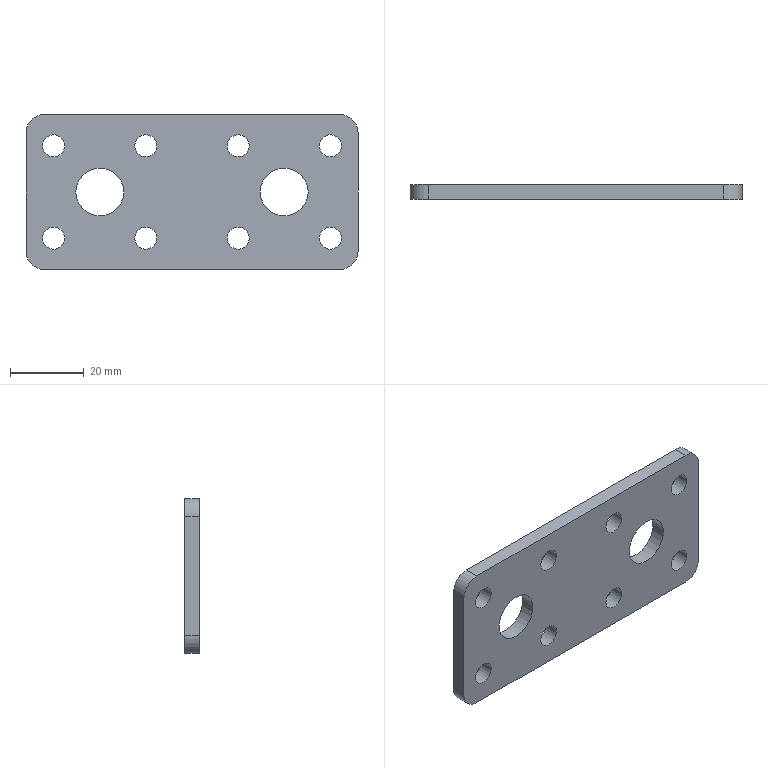Component | SolidWorks | ConnectingPlate(No.9)-3 | 1 solid | 30 faces | box 90 x 4 x 42 mm | volume 13068 mm3 | cylinder 24 | plane 6 | commonest cylinder face diameters 6 x16 13 x4 10 x4 | material Plain Carbon Steel
STEP:
#1=CARTESIAN_POINT('',(12.185,-14.764,-0.4921));
#2=VERTEX_POINT('',#1);
#3=CARTESIAN_POINT('',(12.421,-14.764,-0.4921));
#4=VERTEX_POINT('',#3);
#5=CARTESIAN_POINT('',(12.303,-14.764,-0.4921));
#6=DIRECTION('',(-0.,1.,0.));
#7=DIRECTION('',(-1.,0.,0.));
#8=AXIS2_PLACEMENT_3D('',#5,#6,#7);
#9=CIRCLE('',#8,0.1181);
#10=EDGE_CURVE('',#2,#4,#9,.T.);
#11=ORIENTED_EDGE('',*,*,#10,.F.);
#12=CARTESIAN_POINT('',(12.185,-14.606,-0.4921));
#13=VERTEX_POINT('',#12);
#14=CARTESIAN_POINT('',(12.185,-14.764,-0.4921));
#15=DIRECTION('',(-0.,1.,0.));
#16=VECTOR('',#15,39.37);
#17=LINE('',#14,#16);
#18=EDGE_CURVE('',#2,#13,#17,.T.);
#19=ORIENTED_EDGE('',*,*,#18,.T.);
#20=CARTESIAN_POINT('',(12.421,-14.606,-0.4921));
#21=VERTEX_POINT('',#20);
#22=CARTESIAN_POINT('',(12.303,-14.606,-0.4921));
#23=DIRECTION('',(-0.,1.,0.));
#24=DIRECTION('',(-1.,0.,0.));
#25=AXIS2_PLACEMENT_3D('',#22,#23,#24);
#26=CIRCLE('',#25,0.1181);
#27=EDGE_CURVE('',#13,#21,#26,.T.);
#28=ORIENTED_EDGE('',*,*,#27,.T.);
#29=CARTESIAN_POINT('',(12.421,-14.764,-0.4921));
#30=DIRECTION('',(-0.,1.,0.));
#31=VECTOR('',#30,39.37);
#32=LINE('',#29,#31);
#33=EDGE_CURVE('',#4,#21,#32,.T.);
#34=ORIENTED_EDGE('',*,*,#33,.F.);
#35=EDGE_LOOP('',(#11,#19,#28,#34));
#36=FACE_OUTER_BOUND('',#35,.T.);
#37=CARTESIAN_POINT('',(12.303,-14.764,-0.4921));
#38=DIRECTION('',(-0.,1.,0.));
#39=DIRECTION('',(1.,0.,-0.));
#40=AXIS2_PLACEMENT_3D('',#37,#38,#39);
#41=CYLINDRICAL_SURFACE('',#40,0.1181);
#42=ADVANCED_FACE('',(#36),#41,.F.);
#43=CARTESIAN_POINT('',(13.169,-14.764,-0.4921));
#44=VERTEX_POINT('',#43);
#45=CARTESIAN_POINT('',(13.406,-14.764,-0.4921));
#46=VERTEX_POINT('',#45);
#47=CARTESIAN_POINT('',(13.287,-14.764,-0.4921));
#48=DIRECTION('',(-0.,1.,0.));
#49=DIRECTION('',(-1.,0.,0.));
#50=AXIS2_PLACEMENT_3D('',#47,#48,#49);
#51=CIRCLE('',#50,0.1181);
#52=EDGE_CURVE('',#44,#46,#51,.T.);
#53=ORIENTED_EDGE('',*,*,#52,.F.);
#54=CARTESIAN_POINT('',(13.169,-14.606,-0.4921));
#55=VERTEX_POINT('',#54);
#56=CARTESIAN_POINT('',(13.169,-14.764,-0.4921));
#57=DIRECTION('',(-0.,1.,0.));
#58=VECTOR('',#57,39.37);
#59=LINE('',#56,#58);
#60=EDGE_CURVE('',#44,#55,#59,.T.);
#61=ORIENTED_EDGE('',*,*,#60,.T.);
#62=CARTESIAN_POINT('',(13.406,-14.606,-0.4921));
#63=VERTEX_POINT('',#62);
#64=CARTESIAN_POINT('',(13.287,-14.606,-0.4921));
#65=DIRECTION('',(-0.,1.,0.));
#66=DIRECTION('',(-1.,0.,0.));
#67=AXIS2_PLACEMENT_3D('',#64,#65,#66);
#68=CIRCLE('',#67,0.1181);
#69=EDGE_CURVE('',#55,#63,#68,.T.);
#70=ORIENTED_EDGE('',*,*,#69,.T.);
#71=CARTESIAN_POINT('',(13.406,-14.764,-0.4921));
#72=DIRECTION('',(-0.,1.,0.));
#73=VECTOR('',#72,39.37);
#74=LINE('',#71,#73);
#75=EDGE_CURVE('',#46,#63,#74,.T.);
#76=ORIENTED_EDGE('',*,*,#75,.F.);
#77=EDGE_LOOP('',(#53,#61,#70,#76));
#78=FACE_OUTER_BOUND('',#77,.T.);
#79=CARTESIAN_POINT('',(13.287,-14.764,-0.4921));
#80=DIRECTION('',(-0.,1.,0.));
#81=DIRECTION('',(1.,0.,-0.));
#82=AXIS2_PLACEMENT_3D('',#79,#80,#81);
#83=CYLINDRICAL_SURFACE('',#82,0.1181);
#84=ADVANCED_FACE('',(#78),#83,.F.);
#85=CARTESIAN_POINT('',(14.154,-14.764,-0.4921));
#86=VERTEX_POINT('',#85);
#87=CARTESIAN_POINT('',(14.39,-14.764,-0.4921));
#88=VERTEX_POINT('',#87);
#89=CARTESIAN_POINT('',(14.272,-14.764,-0.4921));
#90=DIRECTION('',(-0.,1.,0.));
#91=DIRECTION('',(-1.,0.,0.));
#92=AXIS2_PLACEMENT_3D('',#89,#90,#91);
#93=CIRCLE('',#92,0.1181);
#94=EDGE_CURVE('',#86,#88,#93,.T.);
#95=ORIENTED_EDGE('',*,*,#94,.F.);
#96=CARTESIAN_POINT('',(14.154,-14.606,-0.4921));
#97=VERTEX_POINT('',#96);
#98=CARTESIAN_POINT('',(14.154,-14.764,-0.4921));
#99=DIRECTION('',(-0.,1.,0.));
#100=VECTOR('',#99,39.37);
#101=LINE('',#98,#100);
#102=EDGE_CURVE('',#86,#97,#101,.T.);
#103=ORIENTED_EDGE('',*,*,#102,.T.);
#104=CARTESIAN_POINT('',(14.39,-14.606,-0.4921));
#105=VERTEX_POINT('',#104);
#106=CARTESIAN_POINT('',(14.272,-14.606,-0.4921));
#107=DIRECTION('',(-0.,1.,0.));
#108=DIRECTION('',(-1.,0.,0.));
#109=AXIS2_PLACEMENT_3D('',#106,#107,#108);
#110=CIRCLE('',#109,0.1181);
#111=EDGE_CURVE('',#97,#105,#110,.T.);
#112=ORIENTED_EDGE('',*,*,#111,.T.);
#113=CARTESIAN_POINT('',(14.39,-14.764,-0.4921));
#114=DIRECTION('',(-0.,1.,0.));
#115=VECTOR('',#114,39.37);
#116=LINE('',#113,#115);
#117=EDGE_CURVE('',#88,#105,#116,.T.);
#118=ORIENTED_EDGE('',*,*,#117,.F.);
#119=EDGE_LOOP('',(#95,#103,#112,#118));
#120=FACE_OUTER_BOUND('',#119,.T.);
#121=CARTESIAN_POINT('',(14.272,-14.764,-0.4921));
#122=DIRECTION('',(-0.,1.,0.));
#123=DIRECTION('',(1.,0.,-0.));
#124=AXIS2_PLACEMENT_3D('',#121,#122,#123);
#125=CYLINDRICAL_SURFACE('',#124,0.1181);
#126=ADVANCED_FACE('',(#120),#125,.F.);
#127=CARTESIAN_POINT('',(15.138,-14.764,-0.4921));
#128=VERTEX_POINT('',#127);
#129=CARTESIAN_POINT('',(15.374,-14.764,-0.4921));
#130=VERTEX_POINT('',#129);
#131=CARTESIAN_POINT('',(15.256,-14.764,-0.4921));
#132=DIRECTION('',(-0.,1.,0.));
#133=DIRECTION('',(-1.,0.,0.));
#134=AXIS2_PLACEMENT_3D('',#131,#132,#133);
#135=CIRCLE('',#134,0.1181);
#136=EDGE_CURVE('',#128,#130,#135,.T.);
#137=ORIENTED_EDGE('',*,*,#136,.F.);
#138=CARTESIAN_POINT('',(15.138,-14.606,-0.4921));
#139=VERTEX_POINT('',#138);
#140=CARTESIAN_POINT('',(15.138,-14.764,-0.4921));
#141=DIRECTION('',(-0.,1.,0.));
#142=VECTOR('',#141,39.37);
#143=LINE('',#140,#142);
#144=EDGE_CURVE('',#128,#139,#143,.T.);
#145=ORIENTED_EDGE('',*,*,#144,.T.);
#146=CARTESIAN_POINT('',(15.374,-14.606,-0.4921));
#147=VERTEX_POINT('',#146);
#148=CARTESIAN_POINT('',(15.256,-14.606,-0.4921));
#149=DIRECTION('',(-0.,1.,0.));
#150=DIRECTION('',(-1.,0.,0.));
#151=AXIS2_PLACEMENT_3D('',#148,#149,#150);
#152=CIRCLE('',#151,0.1181);
#153=EDGE_CURVE('',#139,#147,#152,.T.);
#154=ORIENTED_EDGE('',*,*,#153,.T.);
#155=CARTESIAN_POINT('',(15.374,-14.764,-0.4921));
#156=DIRECTION('',(-0.,1.,0.));
#157=VECTOR('',#156,39.37);
#158=LINE('',#155,#157);
#159=EDGE_CURVE('',#130,#147,#158,.T.);
#160=ORIENTED_EDGE('',*,*,#159,.F.);
#161=EDGE_LOOP('',(#137,#145,#154,#160));
#162=FACE_OUTER_BOUND('',#161,.T.);
#163=CARTESIAN_POINT('',(15.256,-14.764,-0.4921));
#164=DIRECTION('',(-0.,1.,0.));
#165=DIRECTION('',(1.,0.,-0.));
#166=AXIS2_PLACEMENT_3D('',#163,#164,#165);
#167=CYLINDRICAL_SURFACE('',#166,0.1181);
#168=ADVANCED_FACE('',(#162),#167,.F.);
#169=CARTESIAN_POINT('',(15.138,-14.764,-1.476));
#170=VERTEX_POINT('',#169);
#171=CARTESIAN_POINT('',(15.374,-14.764,-1.476));
#172=VERTEX_POINT('',#171);
#173=CARTESIAN_POINT('',(15.256,-14.764,-1.476));
#174=DIRECTION('',(-0.,1.,0.));
#175=DIRECTION('',(1.,0.,0.));
#176=AXIS2_PLACEMENT_3D('',#173,#174,#175);
#177=CIRCLE('',#176,0.1181);
#178=EDGE_CURVE('',#170,#172,#177,.T.);
#179=ORIENTED_EDGE('',*,*,#178,.F.);
#180=CARTESIAN_POINT('',(15.138,-14.606,-1.476));
#181=VERTEX_POINT('',#180);
#182=CARTESIAN_POINT('',(15.138,-14.764,-1.476));
#183=DIRECTION('',(-0.,1.,0.));
#184=VECTOR('',#183,39.37);
#185=LINE('',#182,#184);
#186=EDGE_CURVE('',#170,#181,#185,.T.);
#187=ORIENTED_EDGE('',*,*,#186,.T.);
#188=CARTESIAN_POINT('',(15.374,-14.606,-1.476));
#189=VERTEX_POINT('',#188);
#190=CARTESIAN_POINT('',(15.256,-14.606,-1.476));
#191=DIRECTION('',(-0.,1.,0.));
#192=DIRECTION('',(1.,0.,0.));
#193=AXIS2_PLACEMENT_3D('',#190,#191,#192);
#194=CIRCLE('',#193,0.1181);
#195=EDGE_CURVE('',#181,#189,#194,.T.);
#196=ORIENTED_EDGE('',*,*,#195,.T.);
#197=CARTESIAN_POINT('',(15.374,-14.764,-1.476));
#198=DIRECTION('',(-0.,1.,0.));
#199=VECTOR('',#198,39.37);
#200=LINE('',#197,#199);
#201=EDGE_CURVE('',#172,#189,#200,.T.);
#202=ORIENTED_EDGE('',*,*,#201,.F.);
#203=EDGE_LOOP('',(#179,#187,#196,#202));
#204=FACE_OUTER_BOUND('',#203,.T.);
#205=CARTESIAN_POINT('',(15.256,-14.764,-1.476));
#206=DIRECTION('',(-0.,1.,0.));
#207=DIRECTION('',(1.,0.,0.));
#208=AXIS2_PLACEMENT_3D('',#205,#206,#207);
#209=CYLINDRICAL_SURFACE('',#208,0.1181);
#210=ADVANCED_FACE('',(#204),#209,.F.);
#211=CARTESIAN_POINT('',(14.154,-14.764,-1.476));
#212=VERTEX_POINT('',#211);
#213=CARTESIAN_POINT('',(14.39,-14.764,-1.476));
#214=VERTEX_POINT('',#213);
#215=CARTESIAN_POINT('',(14.272,-14.764,-1.476));
#216=DIRECTION('',(-0.,1.,0.));
#217=DIRECTION('',(1.,0.,0.));
#218=AXIS2_PLACEMENT_3D('',#215,#216,#217);
#219=CIRCLE('',#218,0.1181);
#220=EDGE_CURVE('',#212,#214,#219,.T.);
#221=ORIENTED_EDGE('',*,*,#220,.F.);
#222=CARTESIAN_POINT('',(14.154,-14.606,-1.476));
#223=VERTEX_POINT('',#222);
#224=CARTESIAN_POINT('',(14.154,-14.764,-1.476));
#225=DIRECTION('',(-0.,1.,0.));
#226=VECTOR('',#225,39.37);
#227=LINE('',#224,#226);
#228=EDGE_CURVE('',#212,#223,#227,.T.);
#229=ORIENTED_EDGE('',*,*,#228,.T.);
#230=CARTESIAN_POINT('',(14.39,-14.606,-1.476));
#231=VERTEX_POINT('',#230);
#232=CARTESIAN_POINT('',(14.272,-14.606,-1.476));
#233=DIRECTION('',(-0.,1.,0.));
#234=DIRECTION('',(1.,0.,0.));
#235=AXIS2_PLACEMENT_3D('',#232,#233,#234);
#236=CIRCLE('',#235,0.1181);
#237=EDGE_CURVE('',#223,#231,#236,.T.);
#238=ORIENTED_EDGE('',*,*,#237,.T.);
#239=CARTESIAN_POINT('',(14.39,-14.764,-1.476));
#240=DIRECTION('',(-0.,1.,0.));
#241=VECTOR('',#240,39.37);
#242=LINE('',#239,#241);
#243=EDGE_CURVE('',#214,#231,#242,.T.);
#244=ORIENTED_EDGE('',*,*,#243,.F.);
#245=EDGE_LOOP('',(#221,#229,#238,#244));
#246=FACE_OUTER_BOUND('',#245,.T.);
#247=CARTESIAN_POINT('',(14.272,-14.764,-1.476));
#248=DIRECTION('',(-0.,1.,0.));
#249=DIRECTION('',(1.,0.,0.));
#250=AXIS2_PLACEMENT_3D('',#247,#248,#249);
#251=CYLINDRICAL_SURFACE('',#250,0.1181);
#252=ADVANCED_FACE('',(#246),#251,.F.);
#253=CARTESIAN_POINT('',(13.169,-14.764,-1.476));
#254=VERTEX_POINT('',#253);
#255=CARTESIAN_POINT('',(13.406,-14.764,-1.476));
#256=VERTEX_POINT('',#255);
#257=CARTESIAN_POINT('',(13.287,-14.764,-1.476));
#258=DIRECTION('',(-0.,1.,0.));
#259=DIRECTION('',(1.,0.,0.));
#260=AXIS2_PLACEMENT_3D('',#257,#258,#259);
#261=CIRCLE('',#260,0.1181);
#262=EDGE_CURVE('',#254,#256,#261,.T.);
#263=ORIENTED_EDGE('',*,*,#262,.F.);
#264=CARTESIAN_POINT('',(13.169,-14.606,-1.476));
#265=VERTEX_POINT('',#264);
#266=CARTESIAN_POINT('',(13.169,-14.764,-1.476));
#267=DIRECTION('',(-0.,1.,0.));
#268=VECTOR('',#267,39.37);
#269=LINE('',#266,#268);
#270=EDGE_CURVE('',#254,#265,#269,.T.);
#271=ORIENTED_EDGE('',*,*,#270,.T.);
#272=CARTESIAN_POINT('',(13.406,-14.606,-1.476));
#273=VERTEX_POINT('',#272);
#274=CARTESIAN_POINT('',(13.287,-14.606,-1.476));
#275=DIRECTION('',(-0.,1.,0.));
#276=DIRECTION('',(1.,0.,0.));
#277=AXIS2_PLACEMENT_3D('',#274,#275,#276);
#278=CIRCLE('',#277,0.1181);
#279=EDGE_CURVE('',#265,#273,#278,.T.);
#280=ORIENTED_EDGE('',*,*,#279,.T.);
#281=CARTESIAN_POINT('',(13.406,-14.764,-1.476));
#282=DIRECTION('',(-0.,1.,0.));
#283=VECTOR('',#282,39.37);
#284=LINE('',#281,#283);
#285=EDGE_CURVE('',#256,#273,#284,.T.);
#286=ORIENTED_EDGE('',*,*,#285,.F.);
#287=EDGE_LOOP('',(#263,#271,#280,#286));
#288=FACE_OUTER_BOUND('',#287,.T.);
#289=CARTESIAN_POINT('',(13.287,-14.764,-1.476));
#290=DIRECTION('',(-0.,1.,0.));
#291=DIRECTION('',(1.,0.,0.));
#292=AXIS2_PLACEMENT_3D('',#289,#290,#291);
#293=CYLINDRICAL_SURFACE('',#292,0.1181);
#294=ADVANCED_FACE('',(#288),#293,.F.);
#295=CARTESIAN_POINT('',(12.185,-14.764,-1.476));
#296=VERTEX_POINT('',#295);
#297=CARTESIAN_POINT('',(12.421,-14.764,-1.476));
#298=VERTEX_POINT('',#297);
#299=CARTESIAN_POINT('',(12.303,-14.764,-1.476));
#300=DIRECTION('',(-0.,1.,0.));
#301=DIRECTION('',(1.,0.,0.));
#302=AXIS2_PLACEMENT_3D('',#299,#300,#301);
#303=CIRCLE('',#302,0.1181);
#304=EDGE_CURVE('',#296,#298,#303,.T.);
#305=ORIENTED_EDGE('',*,*,#304,.F.);
#306=CARTESIAN_POINT('',(12.185,-14.606,-1.476));
#307=VERTEX_POINT('',#306);
#308=CARTESIAN_POINT('',(12.185,-14.764,-1.476));
#309=DIRECTION('',(-0.,1.,0.));
#310=VECTOR('',#309,39.37);
#311=LINE('',#308,#310);
#312=EDGE_CURVE('',#296,#307,#311,.T.);
#313=ORIENTED_EDGE('',*,*,#312,.T.);
#314=CARTESIAN_POINT('',(12.421,-14.606,-1.476));
#315=VERTEX_POINT('',#314);
#316=CARTESIAN_POINT('',(12.303,-14.606,-1.476));
#317=DIRECTION('',(-0.,1.,0.));
#318=DIRECTION('',(1.,0.,0.));
#319=AXIS2_PLACEMENT_3D('',#316,#317,#318);
#320=CIRCLE('',#319,0.1181);
#321=EDGE_CURVE('',#307,#315,#320,.T.);
#322=ORIENTED_EDGE('',*,*,#321,.T.);
#323=CARTESIAN_POINT('',(12.421,-14.764,-1.476));
#324=DIRECTION('',(-0.,1.,0.));
#325=VECTOR('',#324,39.37);
#326=LINE('',#323,#325);
#327=EDGE_CURVE('',#298,#315,#326,.T.);
#328=ORIENTED_EDGE('',*,*,#327,.F.);
#329=EDGE_LOOP('',(#305,#313,#322,#328));
#330=FACE_OUTER_BOUND('',#329,.T.);
#331=CARTESIAN_POINT('',(12.303,-14.764,-1.476));
#332=DIRECTION('',(-0.,1.,0.));
#333=DIRECTION('',(1.,0.,0.));
#334=AXIS2_PLACEMENT_3D('',#331,#332,#333);
#335=CYLINDRICAL_SURFACE('',#334,0.1181);
#336=ADVANCED_FACE('',(#330),#335,.F.);
#337=CARTESIAN_POINT('',(14.508,-14.764,-0.9843));
#338=VERTEX_POINT('',#337);
#339=CARTESIAN_POINT('',(15.02,-14.764,-0.9843));
#340=VERTEX_POINT('',#339);
#341=CARTESIAN_POINT('',(14.764,-14.764,-0.9843));
#342=DIRECTION('',(-0.,1.,0.));
#343=DIRECTION('',(-1.,0.,0.));
#344=AXIS2_PLACEMENT_3D('',#341,#342,#343);
#345=CIRCLE('',#344,0.2559);
#346=EDGE_CURVE('',#338,#340,#345,.T.);
#347=ORIENTED_EDGE('',*,*,#346,.F.);
#348=CARTESIAN_POINT('',(14.508,-14.606,-0.9843));
#349=VERTEX_POINT('',#348);
#350=CARTESIAN_POINT('',(14.508,-14.764,-0.9843));
#351=DIRECTION('',(-0.,1.,0.));
#352=VECTOR('',#351,39.37);
#353=LINE('',#350,#352);
#354=EDGE_CURVE('',#338,#349,#353,.T.);
#355=ORIENTED_EDGE('',*,*,#354,.T.);
#356=CARTESIAN_POINT('',(15.02,-14.606,-0.9843));
#357=VERTEX_POINT('',#356);
#358=CARTESIAN_POINT('',(14.764,-14.606,-0.9843));
#359=DIRECTION('',(-0.,1.,0.));
#360=DIRECTION('',(-1.,0.,0.));
#361=AXIS2_PLACEMENT_3D('',#358,#359,#360);
#362=CIRCLE('',#361,0.2559);
#363=EDGE_CURVE('',#349,#357,#362,.T.);
#364=ORIENTED_EDGE('',*,*,#363,.T.);
#365=CARTESIAN_POINT('',(15.02,-14.764,-0.9843));
#366=DIRECTION('',(-0.,1.,0.));
#367=VECTOR('',#366,39.37);
#368=LINE('',#365,#367);
#369=EDGE_CURVE('',#340,#357,#368,.T.);
#370=ORIENTED_EDGE('',*,*,#369,.F.);
#371=EDGE_LOOP('',(#347,#355,#364,#370));
#372=FACE_OUTER_BOUND('',#371,.T.);
#373=CARTESIAN_POINT('',(14.764,-14.764,-0.9843));
#374=DIRECTION('',(-0.,1.,0.));
#375=DIRECTION('',(1.,0.,-0.));
#376=AXIS2_PLACEMENT_3D('',#373,#374,#375);
#377=CYLINDRICAL_SURFACE('',#376,0.2559);
#378=ADVANCED_FACE('',(#372),#377,.F.);
#379=CARTESIAN_POINT('',(12.539,-14.764,-0.9843));
#380=VERTEX_POINT('',#379);
#381=CARTESIAN_POINT('',(13.051,-14.764,-0.9843));
#382=VERTEX_POINT('',#381);
#383=CARTESIAN_POINT('',(12.795,-14.764,-0.9843));
#384=DIRECTION('',(-0.,1.,0.));
#385=DIRECTION('',(1.,0.,-0.));
#386=AXIS2_PLACEMENT_3D('',#383,#384,#385);
#387=CIRCLE('',#386,0.2559);
#388=EDGE_CURVE('',#380,#382,#387,.T.);
#389=ORIENTED_EDGE('',*,*,#388,.F.);
#390=CARTESIAN_POINT('',(12.539,-14.606,-0.9843));
#391=VERTEX_POINT('',#390);
#392=CARTESIAN_POINT('',(12.539,-14.764,-0.9843));
#393=DIRECTION('',(-0.,1.,0.));
#394=VECTOR('',#393,39.37);
#395=LINE('',#392,#394);
#396=EDGE_CURVE('',#380,#391,#395,.T.);
#397=ORIENTED_EDGE('',*,*,#396,.T.);
#398=CARTESIAN_POINT('',(13.051,-14.606,-0.9843));
#399=VERTEX_POINT('',#398);
#400=CARTESIAN_POINT('',(12.795,-14.606,-0.9843));
#401=DIRECTION('',(-0.,1.,0.));
#402=DIRECTION('',(1.,0.,-0.));
#403=AXIS2_PLACEMENT_3D('',#400,#401,#402);
#404=CIRCLE('',#403,0.2559);
#405=EDGE_CURVE('',#391,#399,#404,.T.);
#406=ORIENTED_EDGE('',*,*,#405,.T.);
#407=CARTESIAN_POINT('',(13.051,-14.764,-0.9843));
#408=DIRECTION('',(-0.,1.,0.));
#409=VECTOR('',#408,39.37);
#410=LINE('',#407,#409);
#411=EDGE_CURVE('',#382,#399,#410,.T.);
#412=ORIENTED_EDGE('',*,*,#411,.F.);
#413=EDGE_LOOP('',(#389,#397,#406,#412));
#414=FACE_OUTER_BOUND('',#413,.T.);
#415=CARTESIAN_POINT('',(12.795,-14.764,-0.9843));
#416=DIRECTION('',(-0.,1.,0.));
#417=DIRECTION('',(1.,0.,-0.));
#418=AXIS2_PLACEMENT_3D('',#415,#416,#417);
#419=CYLINDRICAL_SURFACE('',#418,0.2559);
#420=ADVANCED_FACE('',(#414),#419,.F.);
#421=CARTESIAN_POINT('',(15.551,-14.606,-0.3543));
#422=VERTEX_POINT('',#421);
#423=CARTESIAN_POINT('',(15.551,-14.606,-1.614));
#424=VERTEX_POINT('',#423);
#425=CARTESIAN_POINT('',(15.551,-14.606,-0.1575));
#426=DIRECTION('',(-0.,0.,-1.));
#427=VECTOR('',#426,39.37);
#428=LINE('',#425,#427);
#429=EDGE_CURVE('',#422,#424,#428,.T.);
#430=ORIENTED_EDGE('',*,*,#429,.F.);
#431=CARTESIAN_POINT('',(15.551,-14.764,-0.3543));
#432=VERTEX_POINT('',#431);
#433=CARTESIAN_POINT('',(15.551,-14.764,-0.3543));
#434=DIRECTION('',(0.,-1.,-0.));
#435=VECTOR('',#434,39.37);
#436=LINE('',#433,#435);
#437=EDGE_CURVE('',#422,#432,#436,.T.);
#438=ORIENTED_EDGE('',*,*,#437,.T.);
#439=CARTESIAN_POINT('',(15.551,-14.764,-1.614));
#440=VERTEX_POINT('',#439);
#441=CARTESIAN_POINT('',(15.551,-14.764,-0.1575));
#442=DIRECTION('',(-0.,0.,-1.));
#443=VECTOR('',#442,39.37);
#444=LINE('',#441,#443);
#445=EDGE_CURVE('',#432,#440,#444,.T.);
#446=ORIENTED_EDGE('',*,*,#445,.T.);
#447=CARTESIAN_POINT('',(15.551,-14.764,-1.614));
#448=DIRECTION('',(-0.,1.,0.));
#449=VECTOR('',#448,39.37);
#450=LINE('',#447,#449);
#451=EDGE_CURVE('',#440,#424,#450,.T.);
#452=ORIENTED_EDGE('',*,*,#451,.T.);
#453=EDGE_LOOP('',(#430,#438,#446,#452));
#454=FACE_OUTER_BOUND('',#453,.T.);
#455=CARTESIAN_POINT('',(15.551,-14.764,-0.1575));
#456=DIRECTION('',(1.,0.,-0.));
#457=DIRECTION('',(0.,-1.,-0.));
#458=AXIS2_PLACEMENT_3D('',#455,#456,#457);
#459=PLANE('',#458);
#460=ADVANCED_FACE('',(#454),#459,.T.);
#461=CARTESIAN_POINT('',(12.205,-14.606,-0.1575));
#462=VERTEX_POINT('',#461);
#463=CARTESIAN_POINT('',(15.354,-14.606,-0.1575));
#464=VERTEX_POINT('',#463);
#465=CARTESIAN_POINT('',(12.008,-14.606,-0.1575));
#466=DIRECTION('',(1.,0.,-0.));
#467=VECTOR('',#466,39.37);
#468=LINE('',#465,#467);
#469=EDGE_CURVE('',#462,#464,#468,.T.);
#470=ORIENTED_EDGE('',*,*,#469,.F.);
#471=CARTESIAN_POINT('',(12.205,-14.764,-0.1575));
#472=VERTEX_POINT('',#471);
#473=CARTESIAN_POINT('',(12.205,-14.764,-0.1575));
#474=DIRECTION('',(0.,-1.,-0.));
#475=VECTOR('',#474,39.37);
#476=LINE('',#473,#475);
#477=EDGE_CURVE('',#462,#472,#476,.T.);
#478=ORIENTED_EDGE('',*,*,#477,.T.);
#479=CARTESIAN_POINT('',(15.354,-14.764,-0.1575));
#480=VERTEX_POINT('',#479);
#481=CARTESIAN_POINT('',(12.008,-14.764,-0.1575));
#482=DIRECTION('',(1.,0.,-0.));
#483=VECTOR('',#482,39.37);
#484=LINE('',#481,#483);
#485=EDGE_CURVE('',#472,#480,#484,.T.);
#486=ORIENTED_EDGE('',*,*,#485,.T.);
#487=CARTESIAN_POINT('',(15.354,-14.764,-0.1575));
#488=DIRECTION('',(-0.,1.,0.));
#489=VECTOR('',#488,39.37);
#490=LINE('',#487,#489);
#491=EDGE_CURVE('',#480,#464,#490,.T.);
#492=ORIENTED_EDGE('',*,*,#491,.T.);
#493=EDGE_LOOP('',(#470,#478,#486,#492));
#494=FACE_OUTER_BOUND('',#493,.T.);
#495=CARTESIAN_POINT('',(12.008,-14.764,-0.1575));
#496=DIRECTION('',(0.,-0.,1.));
#497=DIRECTION('',(0.,-1.,-0.));
#498=AXIS2_PLACEMENT_3D('',#495,#496,#497);
#499=PLANE('',#498);
#500=ADVANCED_FACE('',(#494),#499,.T.);
#501=CARTESIAN_POINT('',(12.008,-14.764,-1.614));
#502=VERTEX_POINT('',#501);
#503=CARTESIAN_POINT('',(12.008,-14.764,-0.3543));
#504=VERTEX_POINT('',#503);
#505=CARTESIAN_POINT('',(12.008,-14.764,-0.1575));
#506=DIRECTION('',(0.,-0.,1.));
#507=VECTOR('',#506,39.37);
#508=LINE('',#505,#507);
#509=EDGE_CURVE('',#502,#504,#508,.T.);
#510=ORIENTED_EDGE('',*,*,#509,.T.);
#511=CARTESIAN_POINT('',(12.008,-14.606,-0.3543));
#512=VERTEX_POINT('',#511);
#513=CARTESIAN_POINT('',(12.008,-14.764,-0.3543));
#514=DIRECTION('',(-0.,1.,0.));
#515=VECTOR('',#514,39.37);
#516=LINE('',#513,#515);
#517=EDGE_CURVE('',#504,#512,#516,.T.);
#518=ORIENTED_EDGE('',*,*,#517,.T.);
#519=CARTESIAN_POINT('',(12.008,-14.606,-1.614));
#520=VERTEX_POINT('',#519);
#521=CARTESIAN_POINT('',(12.008,-14.606,-0.1575));
#522=DIRECTION('',(0.,-0.,1.));
#523=VECTOR('',#522,39.37);
#524=LINE('',#521,#523);
#525=EDGE_CURVE('',#520,#512,#524,.T.);
#526=ORIENTED_EDGE('',*,*,#525,.F.);
#527=CARTESIAN_POINT('',(12.008,-14.764,-1.614));
#528=DIRECTION('',(0.,-1.,-0.));
#529=VECTOR('',#528,39.37);
#530=LINE('',#527,#529);
#531=EDGE_CURVE('',#520,#502,#530,.T.);
#532=ORIENTED_EDGE('',*,*,#531,.T.);
#533=EDGE_LOOP('',(#510,#518,#526,#532));
#534=FACE_OUTER_BOUND('',#533,.T.);
#535=CARTESIAN_POINT('',(12.008,-14.764,-0.1575));
#536=DIRECTION('',(-1.,-0.,0.));
#537=DIRECTION('',(-0.,1.,0.));
#538=AXIS2_PLACEMENT_3D('',#535,#536,#537);
#539=PLANE('',#538);
#540=ADVANCED_FACE('',(#534),#539,.T.);
#541=CARTESIAN_POINT('',(15.354,-14.764,-1.811));
#542=VERTEX_POINT('',#541);
#543=CARTESIAN_POINT('',(12.205,-14.764,-1.811));
#544=VERTEX_POINT('',#543);
#545=CARTESIAN_POINT('',(12.008,-14.764,-1.811));
#546=DIRECTION('',(-1.,-0.,0.));
#547=VECTOR('',#546,39.37);
#548=LINE('',#545,#547);
#549=EDGE_CURVE('',#542,#544,#548,.T.);
#550=ORIENTED_EDGE('',*,*,#549,.T.);
#551=CARTESIAN_POINT('',(12.205,-14.606,-1.811));
#552=VERTEX_POINT('',#551);
#553=CARTESIAN_POINT('',(12.205,-14.764,-1.811));
#554=DIRECTION('',(-0.,1.,0.));
#555=VECTOR('',#554,39.37);
#556=LINE('',#553,#555);
#557=EDGE_CURVE('',#544,#552,#556,.T.);
#558=ORIENTED_EDGE('',*,*,#557,.T.);
#559=CARTESIAN_POINT('',(15.354,-14.606,-1.811));
#560=VERTEX_POINT('',#559);
#561=CARTESIAN_POINT('',(12.008,-14.606,-1.811));
#562=DIRECTION('',(-1.,-0.,0.));
#563=VECTOR('',#562,39.37);
#564=LINE('',#561,#563);
#565=EDGE_CURVE('',#560,#552,#564,.T.);
#566=ORIENTED_EDGE('',*,*,#565,.F.);
#567=CARTESIAN_POINT('',(15.354,-14.764,-1.811));
#568=DIRECTION('',(0.,-1.,-0.));
#569=VECTOR('',#568,39.37);
#570=LINE('',#567,#569);
#571=EDGE_CURVE('',#560,#542,#570,.T.);
#572=ORIENTED_EDGE('',*,*,#571,.T.);
#573=EDGE_LOOP('',(#550,#558,#566,#572));
#574=FACE_OUTER_BOUND('',#573,.T.);
#575=CARTESIAN_POINT('',(12.008,-14.764,-1.811));
#576=DIRECTION('',(-0.,0.,-1.));
#577=DIRECTION('',(-0.,1.,0.));
#578=AXIS2_PLACEMENT_3D('',#575,#576,#577);
#579=PLANE('',#578);
#580=ADVANCED_FACE('',(#574),#579,.T.);
#581=CARTESIAN_POINT('',(12.303,-14.764,-0.4921));
#582=DIRECTION('',(-0.,1.,0.));
#583=DIRECTION('',(-1.,0.,0.));
#584=AXIS2_PLACEMENT_3D('',#581,#582,#583);
#585=CIRCLE('',#584,0.1181);
#586=EDGE_CURVE('',#4,#2,#585,.T.);
#587=ORIENTED_EDGE('',*,*,#586,.T.);
#588=ORIENTED_EDGE('',*,*,#10,.T.);
#589=EDGE_LOOP('',(#587,#588));
#590=FACE_BOUND('',#589,.T.);
#591=CARTESIAN_POINT('',(13.287,-14.764,-0.4921));
#592=DIRECTION('',(-0.,1.,0.));
#593=DIRECTION('',(-1.,0.,0.));
#594=AXIS2_PLACEMENT_3D('',#591,#592,#593);
#595=CIRCLE('',#594,0.1181);
#596=EDGE_CURVE('',#46,#44,#595,.T.);
#597=ORIENTED_EDGE('',*,*,#596,.T.);
#598=ORIENTED_EDGE('',*,*,#52,.T.);
#599=EDGE_LOOP('',(#597,#598));
#600=FACE_BOUND('',#599,.T.);
#601=CARTESIAN_POINT('',(14.272,-14.764,-0.4921));
#602=DIRECTION('',(-0.,1.,0.));
#603=DIRECTION('',(-1.,0.,0.));
#604=AXIS2_PLACEMENT_3D('',#601,#602,#603);
#605=CIRCLE('',#604,0.1181);
#606=EDGE_CURVE('',#88,#86,#605,.T.);
#607=ORIENTED_EDGE('',*,*,#606,.T.);
#608=ORIENTED_EDGE('',*,*,#94,.T.);
#609=EDGE_LOOP('',(#607,#608));
#610=FACE_BOUND('',#609,.T.);
#611=CARTESIAN_POINT('',(15.256,-14.764,-0.4921));
#612=DIRECTION('',(-0.,1.,0.));
#613=DIRECTION('',(-1.,0.,0.));
#614=AXIS2_PLACEMENT_3D('',#611,#612,#613);
#615=CIRCLE('',#614,0.1181);
#616=EDGE_CURVE('',#130,#128,#615,.T.);
#617=ORIENTED_EDGE('',*,*,#616,.T.);
#618=ORIENTED_EDGE('',*,*,#136,.T.);
#619=EDGE_LOOP('',(#617,#618));
#620=FACE_BOUND('',#619,.T.);
#621=CARTESIAN_POINT('',(15.256,-14.764,-1.476));
#622=DIRECTION('',(-0.,1.,0.));
#623=DIRECTION('',(1.,0.,0.));
#624=AXIS2_PLACEMENT_3D('',#621,#622,#623);
#625=CIRCLE('',#624,0.1181);
#626=EDGE_CURVE('',#172,#170,#625,.T.);
#627=ORIENTED_EDGE('',*,*,#626,.T.);
#628=ORIENTED_EDGE('',*,*,#178,.T.);
#629=EDGE_LOOP('',(#627,#628));
#630=FACE_BOUND('',#629,.T.);
#631=CARTESIAN_POINT('',(14.272,-14.764,-1.476));
#632=DIRECTION('',(-0.,1.,0.));
#633=DIRECTION('',(1.,0.,0.));
#634=AXIS2_PLACEMENT_3D('',#631,#632,#633);
#635=CIRCLE('',#634,0.1181);
#636=EDGE_CURVE('',#214,#212,#635,.T.);
#637=ORIENTED_EDGE('',*,*,#636,.T.);
#638=ORIENTED_EDGE('',*,*,#220,.T.);
#639=EDGE_LOOP('',(#637,#638));
#640=FACE_BOUND('',#639,.T.);
#641=CARTESIAN_POINT('',(13.287,-14.764,-1.476));
#642=DIRECTION('',(-0.,1.,0.));
#643=DIRECTION('',(1.,0.,0.));
#644=AXIS2_PLACEMENT_3D('',#641,#642,#643);
#645=CIRCLE('',#644,0.1181);
#646=EDGE_CURVE('',#256,#254,#645,.T.);
#647=ORIENTED_EDGE('',*,*,#646,.T.);
#648=ORIENTED_EDGE('',*,*,#262,.T.);
#649=EDGE_LOOP('',(#647,#648));
#650=FACE_BOUND('',#649,.T.);
#651=CARTESIAN_POINT('',(12.303,-14.764,-1.476));
#652=DIRECTION('',(-0.,1.,0.));
#653=DIRECTION('',(1.,0.,0.));
#654=AXIS2_PLACEMENT_3D('',#651,#652,#653);
#655=CIRCLE('',#654,0.1181);
#656=EDGE_CURVE('',#298,#296,#655,.T.);
#657=ORIENTED_EDGE('',*,*,#656,.T.);
#658=ORIENTED_EDGE('',*,*,#304,.T.);
#659=EDGE_LOOP('',(#657,#658));
#660=FACE_BOUND('',#659,.T.);
#661=CARTESIAN_POINT('',(14.764,-14.764,-0.9843));
#662=DIRECTION('',(-0.,1.,0.));
#663=DIRECTION('',(-1.,0.,0.));
#664=AXIS2_PLACEMENT_3D('',#661,#662,#663);
#665=CIRCLE('',#664,0.2559);
#666=EDGE_CURVE('',#340,#338,#665,.T.);
#667=ORIENTED_EDGE('',*,*,#666,.T.);
#668=ORIENTED_EDGE('',*,*,#346,.T.);
#669=EDGE_LOOP('',(#667,#668));
#670=FACE_BOUND('',#669,.T.);
#671=CARTESIAN_POINT('',(12.795,-14.764,-0.9843));
#672=DIRECTION('',(-0.,1.,0.));
#673=DIRECTION('',(1.,0.,-0.));
#674=AXIS2_PLACEMENT_3D('',#671,#672,#673);
#675=CIRCLE('',#674,0.2559);
#676=EDGE_CURVE('',#382,#380,#675,.T.);
#677=ORIENTED_EDGE('',*,*,#676,.T.);
#678=ORIENTED_EDGE('',*,*,#388,.T.);
#679=EDGE_LOOP('',(#677,#678));
#680=FACE_BOUND('',#679,.T.);
#681=ORIENTED_EDGE('',*,*,#485,.F.);
#682=CARTESIAN_POINT('',(12.205,-14.764,-0.3543));
#683=DIRECTION('',(0.,-1.,-0.));
#684=DIRECTION('',(-1.,0.,0.));
#685=AXIS2_PLACEMENT_3D('',#682,#683,#684);
#686=CIRCLE('',#685,0.1969);
#687=EDGE_CURVE('',#472,#504,#686,.T.);
#688=ORIENTED_EDGE('',*,*,#687,.T.);
#689=ORIENTED_EDGE('',*,*,#509,.F.);
#690=CARTESIAN_POINT('',(12.205,-14.764,-1.614));
#691=DIRECTION('',(0.,-1.,-0.));
#692=DIRECTION('',(-1.,0.,0.));
#693=AXIS2_PLACEMENT_3D('',#690,#691,#692);
#694=CIRCLE('',#693,0.1969);
#695=EDGE_CURVE('',#502,#544,#694,.T.);
#696=ORIENTED_EDGE('',*,*,#695,.T.);
#697=ORIENTED_EDGE('',*,*,#549,.F.);
#698=CARTESIAN_POINT('',(15.354,-14.764,-1.614));
#699=DIRECTION('',(0.,-1.,-0.));
#700=DIRECTION('',(-1.,0.,0.));
#701=AXIS2_PLACEMENT_3D('',#698,#699,#700);
#702=CIRCLE('',#701,0.1969);
#703=EDGE_CURVE('',#542,#440,#702,.T.);
#704=ORIENTED_EDGE('',*,*,#703,.T.);
#705=ORIENTED_EDGE('',*,*,#445,.F.);
#706=CARTESIAN_POINT('',(15.354,-14.764,-0.3543));
#707=DIRECTION('',(0.,-1.,-0.));
#708=DIRECTION('',(-1.,0.,0.));
#709=AXIS2_PLACEMENT_3D('',#706,#707,#708);
#710=CIRCLE('',#709,0.1969);
#711=EDGE_CURVE('',#432,#480,#710,.T.);
#712=ORIENTED_EDGE('',*,*,#711,.T.);
#713=EDGE_LOOP('',(#681,#688,#689,#696,#697,#704,#705,#712));
#714=FACE_OUTER_BOUND('',#713,.T.);
#715=CARTESIAN_POINT('',(15.551,-14.764,-1.811));
#716=DIRECTION('',(0.,-1.,-0.));
#717=DIRECTION('',(-1.,-0.,0.));
#718=AXIS2_PLACEMENT_3D('',#715,#716,#717);
#719=PLANE('',#718);
#720=ADVANCED_FACE('',(#590,#600,#610,#620,#630,#640,#650,#660,#670,#680,#714),#719,.T.);
#721=CARTESIAN_POINT('',(12.303,-14.606,-0.4921));
#722=DIRECTION('',(-0.,1.,0.));
#723=DIRECTION('',(-1.,0.,0.));
#724=AXIS2_PLACEMENT_3D('',#721,#722,#723);
#725=CIRCLE('',#724,0.1181);
#726=EDGE_CURVE('',#21,#13,#725,.T.);
#727=ORIENTED_EDGE('',*,*,#726,.F.);
#728=ORIENTED_EDGE('',*,*,#27,.F.);
#729=EDGE_LOOP('',(#727,#728));
#730=FACE_BOUND('',#729,.T.);
#731=CARTESIAN_POINT('',(13.287,-14.606,-0.4921));
#732=DIRECTION('',(-0.,1.,0.));
#733=DIRECTION('',(-1.,0.,0.));
#734=AXIS2_PLACEMENT_3D('',#731,#732,#733);
#735=CIRCLE('',#734,0.1181);
#736=EDGE_CURVE('',#63,#55,#735,.T.);
#737=ORIENTED_EDGE('',*,*,#736,.F.);
#738=ORIENTED_EDGE('',*,*,#69,.F.);
#739=EDGE_LOOP('',(#737,#738));
#740=FACE_BOUND('',#739,.T.);
#741=CARTESIAN_POINT('',(14.272,-14.606,-0.4921));
#742=DIRECTION('',(-0.,1.,0.));
#743=DIRECTION('',(-1.,0.,0.));
#744=AXIS2_PLACEMENT_3D('',#741,#742,#743);
#745=CIRCLE('',#744,0.1181);
#746=EDGE_CURVE('',#105,#97,#745,.T.);
#747=ORIENTED_EDGE('',*,*,#746,.F.);
#748=ORIENTED_EDGE('',*,*,#111,.F.);
#749=EDGE_LOOP('',(#747,#748));
#750=FACE_BOUND('',#749,.T.);
#751=CARTESIAN_POINT('',(15.256,-14.606,-0.4921));
#752=DIRECTION('',(-0.,1.,0.));
#753=DIRECTION('',(-1.,0.,0.));
#754=AXIS2_PLACEMENT_3D('',#751,#752,#753);
#755=CIRCLE('',#754,0.1181);
#756=EDGE_CURVE('',#147,#139,#755,.T.);
#757=ORIENTED_EDGE('',*,*,#756,.F.);
#758=ORIENTED_EDGE('',*,*,#153,.F.);
#759=EDGE_LOOP('',(#757,#758));
#760=FACE_BOUND('',#759,.T.);
#761=CARTESIAN_POINT('',(15.256,-14.606,-1.476));
#762=DIRECTION('',(-0.,1.,0.));
#763=DIRECTION('',(1.,0.,0.));
#764=AXIS2_PLACEMENT_3D('',#761,#762,#763);
#765=CIRCLE('',#764,0.1181);
#766=EDGE_CURVE('',#189,#181,#765,.T.);
#767=ORIENTED_EDGE('',*,*,#766,.F.);
#768=ORIENTED_EDGE('',*,*,#195,.F.);
#769=EDGE_LOOP('',(#767,#768));
#770=FACE_BOUND('',#769,.T.);
#771=CARTESIAN_POINT('',(14.272,-14.606,-1.476));
#772=DIRECTION('',(-0.,1.,0.));
#773=DIRECTION('',(1.,0.,0.));
#774=AXIS2_PLACEMENT_3D('',#771,#772,#773);
#775=CIRCLE('',#774,0.1181);
#776=EDGE_CURVE('',#231,#223,#775,.T.);
#777=ORIENTED_EDGE('',*,*,#776,.F.);
#778=ORIENTED_EDGE('',*,*,#237,.F.);
#779=EDGE_LOOP('',(#777,#778));
#780=FACE_BOUND('',#779,.T.);
#781=CARTESIAN_POINT('',(13.287,-14.606,-1.476));
#782=DIRECTION('',(-0.,1.,0.));
#783=DIRECTION('',(1.,0.,0.));
#784=AXIS2_PLACEMENT_3D('',#781,#782,#783);
#785=CIRCLE('',#784,0.1181);
#786=EDGE_CURVE('',#273,#265,#785,.T.);
#787=ORIENTED_EDGE('',*,*,#786,.F.);
#788=ORIENTED_EDGE('',*,*,#279,.F.);
#789=EDGE_LOOP('',(#787,#788));
#790=FACE_BOUND('',#789,.T.);
#791=CARTESIAN_POINT('',(12.303,-14.606,-1.476));
#792=DIRECTION('',(-0.,1.,0.));
#793=DIRECTION('',(1.,0.,0.));
#794=AXIS2_PLACEMENT_3D('',#791,#792,#793);
#795=CIRCLE('',#794,0.1181);
#796=EDGE_CURVE('',#315,#307,#795,.T.);
#797=ORIENTED_EDGE('',*,*,#796,.F.);
#798=ORIENTED_EDGE('',*,*,#321,.F.);
#799=EDGE_LOOP('',(#797,#798));
#800=FACE_BOUND('',#799,.T.);
#801=CARTESIAN_POINT('',(14.764,-14.606,-0.9843));
#802=DIRECTION('',(-0.,1.,0.));
#803=DIRECTION('',(-1.,0.,0.));
#804=AXIS2_PLACEMENT_3D('',#801,#802,#803);
#805=CIRCLE('',#804,0.2559);
#806=EDGE_CURVE('',#357,#349,#805,.T.);
#807=ORIENTED_EDGE('',*,*,#806,.F.);
#808=ORIENTED_EDGE('',*,*,#363,.F.);
#809=EDGE_LOOP('',(#807,#808));
#810=FACE_BOUND('',#809,.T.);
#811=CARTESIAN_POINT('',(12.795,-14.606,-0.9843));
#812=DIRECTION('',(-0.,1.,0.));
#813=DIRECTION('',(1.,0.,-0.));
#814=AXIS2_PLACEMENT_3D('',#811,#812,#813);
#815=CIRCLE('',#814,0.2559);
#816=EDGE_CURVE('',#399,#391,#815,.T.);
#817=ORIENTED_EDGE('',*,*,#816,.F.);
#818=ORIENTED_EDGE('',*,*,#405,.F.);
#819=EDGE_LOOP('',(#817,#818));
#820=FACE_BOUND('',#819,.T.);
#821=ORIENTED_EDGE('',*,*,#525,.T.);
#822=CARTESIAN_POINT('',(12.205,-14.606,-0.3543));
#823=DIRECTION('',(-0.,1.,0.));
#824=DIRECTION('',(-1.,0.,0.));
#825=AXIS2_PLACEMENT_3D('',#822,#823,#824);
#826=CIRCLE('',#825,0.1969);
#827=EDGE_CURVE('',#512,#462,#826,.T.);
#828=ORIENTED_EDGE('',*,*,#827,.T.);
#829=ORIENTED_EDGE('',*,*,#469,.T.);
#830=CARTESIAN_POINT('',(15.354,-14.606,-0.3543));
#831=DIRECTION('',(-0.,1.,0.));
#832=DIRECTION('',(-1.,0.,0.));
#833=AXIS2_PLACEMENT_3D('',#830,#831,#832);
#834=CIRCLE('',#833,0.1969);
#835=EDGE_CURVE('',#464,#422,#834,.T.);
#836=ORIENTED_EDGE('',*,*,#835,.T.);
#837=ORIENTED_EDGE('',*,*,#429,.T.);
#838=CARTESIAN_POINT('',(15.354,-14.606,-1.614));
#839=DIRECTION('',(-0.,1.,0.));
#840=DIRECTION('',(-1.,0.,0.));
#841=AXIS2_PLACEMENT_3D('',#838,#839,#840);
#842=CIRCLE('',#841,0.1969);
#843=EDGE_CURVE('',#424,#560,#842,.T.);
#844=ORIENTED_EDGE('',*,*,#843,.T.);
#845=ORIENTED_EDGE('',*,*,#565,.T.);
#846=CARTESIAN_POINT('',(12.205,-14.606,-1.614));
#847=DIRECTION('',(-0.,1.,0.));
#848=DIRECTION('',(-1.,0.,-0.));
#849=AXIS2_PLACEMENT_3D('',#846,#847,#848);
#850=CIRCLE('',#849,0.1969);
#851=EDGE_CURVE('',#552,#520,#850,.T.);
#852=ORIENTED_EDGE('',*,*,#851,.T.);
#853=EDGE_LOOP('',(#821,#828,#829,#836,#837,#844,#845,#852));
#854=FACE_OUTER_BOUND('',#853,.T.);
#855=CARTESIAN_POINT('',(15.551,-14.606,-1.811));
#856=DIRECTION('',(0.,-1.,-0.));
#857=DIRECTION('',(-1.,-0.,0.));
#858=AXIS2_PLACEMENT_3D('',#855,#856,#857);
#859=PLANE('',#858);
#860=ADVANCED_FACE('',(#730,#740,#750,#760,#770,#780,#790,#800,#810,#820,#854),#859,.F.);
#861=ORIENTED_EDGE('',*,*,#396,.F.);
#862=ORIENTED_EDGE('',*,*,#676,.F.);
#863=ORIENTED_EDGE('',*,*,#411,.T.);
#864=ORIENTED_EDGE('',*,*,#816,.T.);
#865=EDGE_LOOP('',(#861,#862,#863,#864));
#866=FACE_OUTER_BOUND('',#865,.T.);
#867=CARTESIAN_POINT('',(12.795,-14.764,-0.9843));
#868=DIRECTION('',(-0.,1.,0.));
#869=DIRECTION('',(1.,0.,-0.));
#870=AXIS2_PLACEMENT_3D('',#867,#868,#869);
#871=CYLINDRICAL_SURFACE('',#870,0.2559);
#872=ADVANCED_FACE('',(#866),#871,.F.);
#873=ORIENTED_EDGE('',*,*,#354,.F.);
#874=ORIENTED_EDGE('',*,*,#666,.F.);
#875=ORIENTED_EDGE('',*,*,#369,.T.);
#876=ORIENTED_EDGE('',*,*,#806,.T.);
#877=EDGE_LOOP('',(#873,#874,#875,#876));
#878=FACE_OUTER_BOUND('',#877,.T.);
#879=CARTESIAN_POINT('',(14.764,-14.764,-0.9843));
#880=DIRECTION('',(-0.,1.,0.));
#881=DIRECTION('',(1.,0.,-0.));
#882=AXIS2_PLACEMENT_3D('',#879,#880,#881);
#883=CYLINDRICAL_SURFACE('',#882,0.2559);
#884=ADVANCED_FACE('',(#878),#883,.F.);
#885=ORIENTED_EDGE('',*,*,#687,.F.);
#886=ORIENTED_EDGE('',*,*,#477,.F.);
#887=ORIENTED_EDGE('',*,*,#827,.F.);
#888=ORIENTED_EDGE('',*,*,#517,.F.);
#889=EDGE_LOOP('',(#885,#886,#887,#888));
#890=FACE_OUTER_BOUND('',#889,.T.);
#891=CARTESIAN_POINT('',(12.205,-14.764,-0.3543));
#892=DIRECTION('',(-0.,1.,0.));
#893=DIRECTION('',(1.,0.,-0.));
#894=AXIS2_PLACEMENT_3D('',#891,#892,#893);
#895=CYLINDRICAL_SURFACE('',#894,0.1969);
#896=ADVANCED_FACE('',(#890),#895,.T.);
#897=ORIENTED_EDGE('',*,*,#695,.F.);
#898=ORIENTED_EDGE('',*,*,#531,.F.);
#899=ORIENTED_EDGE('',*,*,#851,.F.);
#900=ORIENTED_EDGE('',*,*,#557,.F.);
#901=EDGE_LOOP('',(#897,#898,#899,#900));
#902=FACE_OUTER_BOUND('',#901,.T.);
#903=CARTESIAN_POINT('',(12.205,-14.764,-1.614));
#904=DIRECTION('',(-0.,1.,0.));
#905=DIRECTION('',(1.,0.,-0.));
#906=AXIS2_PLACEMENT_3D('',#903,#904,#905);
#907=CYLINDRICAL_SURFACE('',#906,0.1969);
#908=ADVANCED_FACE('',(#902),#907,.T.);
#909=ORIENTED_EDGE('',*,*,#711,.F.);
#910=ORIENTED_EDGE('',*,*,#437,.F.);
#911=ORIENTED_EDGE('',*,*,#835,.F.);
#912=ORIENTED_EDGE('',*,*,#491,.F.);
#913=EDGE_LOOP('',(#909,#910,#911,#912));
#914=FACE_OUTER_BOUND('',#913,.T.);
#915=CARTESIAN_POINT('',(15.354,-14.764,-0.3543));
#916=DIRECTION('',(-0.,1.,0.));
#917=DIRECTION('',(1.,0.,-0.));
#918=AXIS2_PLACEMENT_3D('',#915,#916,#917);
#919=CYLINDRICAL_SURFACE('',#918,0.1969);
#920=ADVANCED_FACE('',(#914),#919,.T.);
#921=ORIENTED_EDGE('',*,*,#703,.F.);
#922=ORIENTED_EDGE('',*,*,#571,.F.);
#923=ORIENTED_EDGE('',*,*,#843,.F.);
#924=ORIENTED_EDGE('',*,*,#451,.F.);
#925=EDGE_LOOP('',(#921,#922,#923,#924));
#926=FACE_OUTER_BOUND('',#925,.T.);
#927=CARTESIAN_POINT('',(15.354,-14.764,-1.614));
#928=DIRECTION('',(-0.,1.,0.));
#929=DIRECTION('',(1.,0.,-0.));
#930=AXIS2_PLACEMENT_3D('',#927,#928,#929);
#931=CYLINDRICAL_SURFACE('',#930,0.1969);
#932=ADVANCED_FACE('',(#926),#931,.T.);
#933=ORIENTED_EDGE('',*,*,#312,.F.);
#934=ORIENTED_EDGE('',*,*,#656,.F.);
#935=ORIENTED_EDGE('',*,*,#327,.T.);
#936=ORIENTED_EDGE('',*,*,#796,.T.);
#937=EDGE_LOOP('',(#933,#934,#935,#936));
#938=FACE_OUTER_BOUND('',#937,.T.);
#939=CARTESIAN_POINT('',(12.303,-14.764,-1.476));
#940=DIRECTION('',(-0.,1.,0.));
#941=DIRECTION('',(1.,0.,0.));
#942=AXIS2_PLACEMENT_3D('',#939,#940,#941);
#943=CYLINDRICAL_SURFACE('',#942,0.1181);
#944=ADVANCED_FACE('',(#938),#943,.F.);
#945=ORIENTED_EDGE('',*,*,#270,.F.);
#946=ORIENTED_EDGE('',*,*,#646,.F.);
#947=ORIENTED_EDGE('',*,*,#285,.T.);
#948=ORIENTED_EDGE('',*,*,#786,.T.);
#949=EDGE_LOOP('',(#945,#946,#947,#948));
#950=FACE_OUTER_BOUND('',#949,.T.);
#951=CARTESIAN_POINT('',(13.287,-14.764,-1.476));
#952=DIRECTION('',(-0.,1.,0.));
#953=DIRECTION('',(1.,0.,0.));
#954=AXIS2_PLACEMENT_3D('',#951,#952,#953);
#955=CYLINDRICAL_SURFACE('',#954,0.1181);
#956=ADVANCED_FACE('',(#950),#955,.F.);
#957=ORIENTED_EDGE('',*,*,#228,.F.);
#958=ORIENTED_EDGE('',*,*,#636,.F.);
#959=ORIENTED_EDGE('',*,*,#243,.T.);
#960=ORIENTED_EDGE('',*,*,#776,.T.);
#961=EDGE_LOOP('',(#957,#958,#959,#960));
#962=FACE_OUTER_BOUND('',#961,.T.);
#963=CARTESIAN_POINT('',(14.272,-14.764,-1.476));
#964=DIRECTION('',(-0.,1.,0.));
#965=DIRECTION('',(1.,0.,0.));
#966=AXIS2_PLACEMENT_3D('',#963,#964,#965);
#967=CYLINDRICAL_SURFACE('',#966,0.1181);
#968=ADVANCED_FACE('',(#962),#967,.F.);
#969=ORIENTED_EDGE('',*,*,#186,.F.);
#970=ORIENTED_EDGE('',*,*,#626,.F.);
#971=ORIENTED_EDGE('',*,*,#201,.T.);
#972=ORIENTED_EDGE('',*,*,#766,.T.);
#973=EDGE_LOOP('',(#969,#970,#971,#972));
#974=FACE_OUTER_BOUND('',#973,.T.);
#975=CARTESIAN_POINT('',(15.256,-14.764,-1.476));
#976=DIRECTION('',(-0.,1.,0.));
#977=DIRECTION('',(1.,0.,0.));
#978=AXIS2_PLACEMENT_3D('',#975,#976,#977);
#979=CYLINDRICAL_SURFACE('',#978,0.1181);
#980=ADVANCED_FACE('',(#974),#979,.F.);
#981=ORIENTED_EDGE('',*,*,#144,.F.);
#982=ORIENTED_EDGE('',*,*,#616,.F.);
#983=ORIENTED_EDGE('',*,*,#159,.T.);
#984=ORIENTED_EDGE('',*,*,#756,.T.);
#985=EDGE_LOOP('',(#981,#982,#983,#984));
#986=FACE_OUTER_BOUND('',#985,.T.);
#987=CARTESIAN_POINT('',(15.256,-14.764,-0.4921));
#988=DIRECTION('',(-0.,1.,0.));
#989=DIRECTION('',(1.,0.,-0.));
#990=AXIS2_PLACEMENT_3D('',#987,#988,#989);
#991=CYLINDRICAL_SURFACE('',#990,0.1181);
#992=ADVANCED_FACE('',(#986),#991,.F.);
#993=ORIENTED_EDGE('',*,*,#102,.F.);
#994=ORIENTED_EDGE('',*,*,#606,.F.);
#995=ORIENTED_EDGE('',*,*,#117,.T.);
#996=ORIENTED_EDGE('',*,*,#746,.T.);
#997=EDGE_LOOP('',(#993,#994,#995,#996));
#998=FACE_OUTER_BOUND('',#997,.T.);
#999=CARTESIAN_POINT('',(14.272,-14.764,-0.4921));
#1000=DIRECTION('',(-0.,1.,0.));
#1001=DIRECTION('',(1.,0.,-0.));
#1002=AXIS2_PLACEMENT_3D('',#999,#1000,#1001);
#1003=CYLINDRICAL_SURFACE('',#1002,0.1181);
#1004=ADVANCED_FACE('',(#998),#1003,.F.);
#1005=ORIENTED_EDGE('',*,*,#60,.F.);
#1006=ORIENTED_EDGE('',*,*,#596,.F.);
#1007=ORIENTED_EDGE('',*,*,#75,.T.);
#1008=ORIENTED_EDGE('',*,*,#736,.T.);
#1009=EDGE_LOOP('',(#1005,#1006,#1007,#1008));
#1010=FACE_OUTER_BOUND('',#1009,.T.);
#1011=CARTESIAN_POINT('',(13.287,-14.764,-0.4921));
#1012=DIRECTION('',(-0.,1.,0.));
#1013=DIRECTION('',(1.,0.,-0.));
#1014=AXIS2_PLACEMENT_3D('',#1011,#1012,#1013);
#1015=CYLINDRICAL_SURFACE('',#1014,0.1181);
#1016=ADVANCED_FACE('',(#1010),#1015,.F.);
#1017=ORIENTED_EDGE('',*,*,#18,.F.);
#1018=ORIENTED_EDGE('',*,*,#586,.F.);
#1019=ORIENTED_EDGE('',*,*,#33,.T.);
#1020=ORIENTED_EDGE('',*,*,#726,.T.);
#1021=EDGE_LOOP('',(#1017,#1018,#1019,#1020));
#1022=FACE_OUTER_BOUND('',#1021,.T.);
#1023=CARTESIAN_POINT('',(12.303,-14.764,-0.4921));
#1024=DIRECTION('',(-0.,1.,0.));
#1025=DIRECTION('',(1.,0.,-0.));
#1026=AXIS2_PLACEMENT_3D('',#1023,#1024,#1025);
#1027=CYLINDRICAL_SURFACE('',#1026,0.1181);
#1028=ADVANCED_FACE('',(#1022),#1027,.F.);
#1029=CLOSED_SHELL('',(#42,#84,#126,#168,#210,#252,#294,#336,#378,#420,#460,#500,#540,#580,#720,#860,#872,#884,#896,#908,#920,#932,#944,#956,#968,#980,#992,#1004,#1016,#1028));
#1030=MANIFOLD_SOLID_BREP('',#1029);
#1031=CARTESIAN_POINT('',(0.,0.,0.));
#1032=DIRECTION('',(0.,0.,1.));
#1033=DIRECTION('',(1.,0.,0.));
#1034=AXIS2_PLACEMENT_3D('',#1031,#1032,#1033);
#1035=(LENGTH_UNIT()NAMED_UNIT(*)SI_UNIT($,.METRE.));
#1036=LENGTH_MEASURE_WITH_UNIT(LENGTH_MEASURE(0.0254),#1035);
#1037=DIMENSIONAL_EXPONENTS(1.,0.,0.,0.,0.,0.,0.);
#1038=(CONVERSION_BASED_UNIT('',#1036)LENGTH_UNIT()NAMED_UNIT(#1037));
#1039=UNCERTAINTY_MEASURE_WITH_UNIT(LENGTH_MEASURE(0.00001),#1038,'','');
#1040=(NAMED_UNIT(*)PLANE_ANGLE_UNIT()SI_UNIT($,.RADIAN.));
#1041=(NAMED_UNIT(*)SI_UNIT($,.STERADIAN.)SOLID_ANGLE_UNIT());
#1042=(GEOMETRIC_REPRESENTATION_CONTEXT(3)GLOBAL_UNCERTAINTY_ASSIGNED_CONTEXT((#1039))GLOBAL_UNIT_ASSIGNED_CONTEXT((#1038,#1040,#1041))REPRESENTATION_CONTEXT('',''));
#1043=ADVANCED_BREP_SHAPE_REPRESENTATION('',(#1030,#1034),#1042);
#1044=COLOUR_RGB('',0.7922,0.8196,0.9333);
#1045=FILL_AREA_STYLE_COLOUR('',#1044);
#1046=FILL_AREA_STYLE('',(#1045));
#1047=SURFACE_STYLE_FILL_AREA(#1046);
#1048=SURFACE_SIDE_STYLE('',(#1047));
#1049=SURFACE_STYLE_USAGE(.BOTH.,#1048);
#1050=PRESENTATION_STYLE_ASSIGNMENT((#1049));
#1051=STYLED_ITEM('',(#1050),#1030);
#1052=(LENGTH_UNIT()NAMED_UNIT(*)SI_UNIT($,.METRE.));
#1053=LENGTH_MEASURE_WITH_UNIT(LENGTH_MEASURE(0.0254),#1052);
#1054=DIMENSIONAL_EXPONENTS(1.,0.,0.,0.,0.,0.,0.);
#1055=(CONVERSION_BASED_UNIT('',#1053)LENGTH_UNIT()NAMED_UNIT(#1054));
#1056=UNCERTAINTY_MEASURE_WITH_UNIT(LENGTH_MEASURE(0.00001),#1055,'','');
#1057=(NAMED_UNIT(*)PLANE_ANGLE_UNIT()SI_UNIT($,.RADIAN.));
#1058=(NAMED_UNIT(*)SI_UNIT($,.STERADIAN.)SOLID_ANGLE_UNIT());
#1059=(GEOMETRIC_REPRESENTATION_CONTEXT(3)GLOBAL_UNCERTAINTY_ASSIGNED_CONTEXT((#1056))GLOBAL_UNIT_ASSIGNED_CONTEXT((#1055,#1057,#1058))REPRESENTATION_CONTEXT('',''));
#1060=MECHANICAL_DESIGN_GEOMETRIC_PRESENTATION_REPRESENTATION('',(#1051),#1059);
#1061=PRESENTATION_LAYER_ASSIGNMENT('','',(#1051));